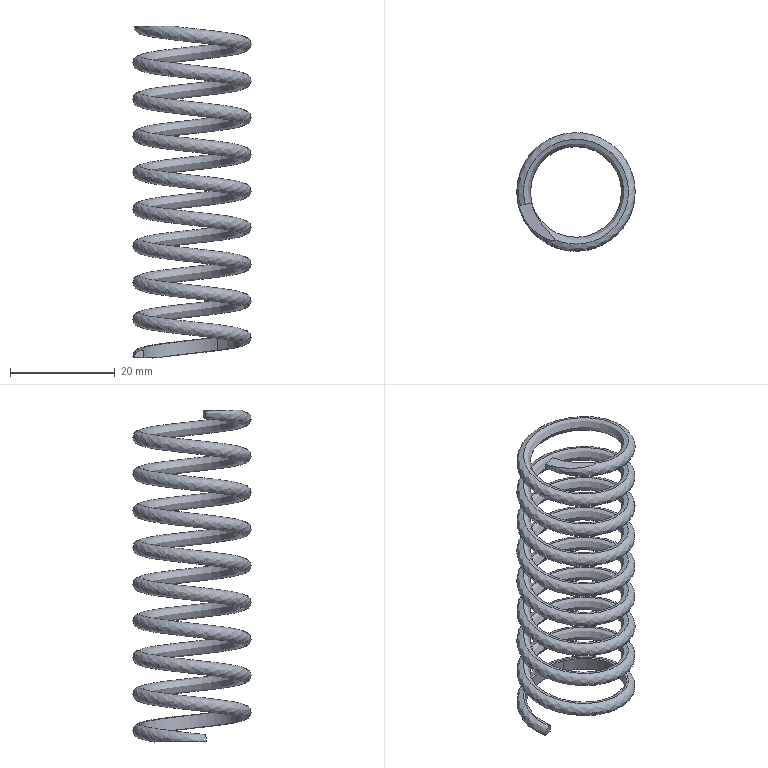Component | SolidWorks | AD12-CompressionSpring.SDPRT-2 | 1 solid | 10 faces | volume 2905 mm3 | plane 5 | cylinder 3 | spline 2 | commonest cylinder face diameters 19.259 x3